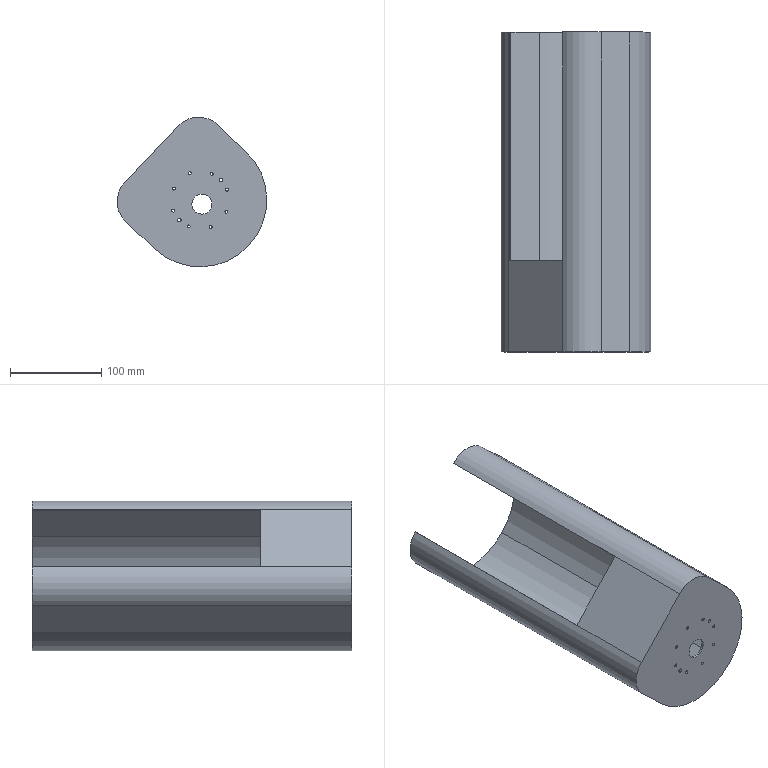Component | SolidWorks | ArmHousing3-1 | 1 solid | 42 faces | box 163.79 x 350 x 163.79 mm | volume 333891 mm3 | cylinder 30 | plane 12 | commonest cylinder face diameters 3.3 x16 4 x4 22 x2 146 x2 142 x2 56 x2 60 x2
build123d program:
from build123d import *

# Parameters (mm, degrees)
BOSS_EXTRUDE1_DEPTH     = 350
FILLET1_R               = 30
SHELL1_T                = -2
BOSS_EXTRUDE2_START     = -2
SKETCH3_R               = 1.65
SKETCH3_R_2             = 2
BOSS_EXTRUDE2_DEPTH     = 2
SKETCH4_W               = 250
SKETCH4_H               = 86
CUT_EXTRUDE1_2_DEPTH    = 2
CUT_EXTRUDE1_DEPTH      = 4
CUT_EXTRUDE1_DEPTH_BACK = 4
SKETCH1_R               = 11


with BuildPart() as part:
    # Sketch2 → Boss-Extrude1 (new body)
    with BuildSketch(Plane.XY):
        with BuildLine():
            Line((90, 148.39), (163, 148.39))
            Line((163, 148.39), (163, 294.39))
            Line((163, 294.39), (90, 294.39))
            ThreePointArc((90, 294.39), (17, 221.39), (90, 148.39))
        make_face()
    extrude(amount=BOSS_EXTRUDE1_DEPTH)

    # Fillet1
    fillet1_edges = [part.edges().sort_by_distance(p)[0] for p in [
        (163, 294.39, 175),
        (163, 148.39, 175),
    ]]
    fillet(fillet1_edges, radius=FILLET1_R)

    # Shell1
    shell1_openings = [part.faces().sort_by_distance(p)[0] for p in [
        (95.582, 221.39, 350),
        (95.582, 221.39, 0),
    ]]
    offset(amount=SHELL1_T, openings=shell1_openings, kind=Kind.INTERSECTION)

    # Sketch3 → Boss-Extrude2 (add)
    with BuildSketch(Plane(origin=(0, 0, 0), x_dir=(-1, 0, 0), z_dir=(0, 0, -1)).offset(BOSS_EXTRUDE2_START)):
        with BuildLine():
            Line((-90, 294.39), (-133, 294.39))
            ThreePointArc((-133, 294.39), (-154.213, 285.603), (-163, 264.39))
            Line((-163, 264.39), (-163, 178.39))
            ThreePointArc((-163, 178.39), (-154.213, 157.177), (-133, 148.39))
            Line((-133, 148.39), (-90, 148.39))
            ThreePointArc((-90, 148.39), (-17, 221.39), (-90, 294.39))
        make_face()
        with Locations((-61.491, 207.992)):
            Circle(SKETCH3_R, mode=Mode.SUBTRACT)
        with Locations((-79.315, 191.757)):
            Circle(SKETCH3_R, mode=Mode.SUBTRACT)
        with Locations((-60.368, 232.075)):
            Circle(SKETCH3_R, mode=Mode.SUBTRACT)
        with Locations((-76.602, 249.899)):
            Circle(SKETCH3_R, mode=Mode.SUBTRACT)
        with Locations((-88.532, 252.856)):
            Circle(SKETCH3_R_2, mode=Mode.SUBTRACT)
        with Locations((-100.685, 251.022)):
            Circle(SKETCH3_R, mode=Mode.SUBTRACT)
        with Locations((-91.468, 189.924)):
            Circle(SKETCH3_R_2, mode=Mode.SUBTRACT)
        with Locations((-103.398, 192.881)):
            Circle(SKETCH3_R, mode=Mode.SUBTRACT)
        with Locations((-119.632, 210.705)):
            Circle(SKETCH3_R, mode=Mode.SUBTRACT)
        with Locations((-118.509, 234.787)):
            Circle(SKETCH3_R, mode=Mode.SUBTRACT)
    extrude(amount=BOSS_EXTRUDE2_DEPTH)

    # Sketch4 → Cut-Extrude1_2 (cut)
    with BuildSketch(Plane(origin=(163, 0, 0), x_dir=(0, 0, -1), z_dir=(1, 0, 0))):
        with Locations((-225, 221.39)):
            Rectangle(SKETCH4_W, SKETCH4_H)
    extrude(amount=-CUT_EXTRUDE1_2_DEPTH, mode=Mode.SUBTRACT)

    # Sketch1 → Cut-Extrude1 (cut, two sides: drawn at the far end of the back side and taken through both)
    with BuildSketch(Plane.XY.offset(-CUT_EXTRUDE1_DEPTH_BACK)):
        with Locations(Location((85.6, 219.613, 0), (0, 0, 180))):
            Circle(SKETCH1_R)
    extrude(amount=CUT_EXTRUDE1_DEPTH + CUT_EXTRUDE1_DEPTH_BACK, mode=Mode.SUBTRACT)


solid = part.part

# Placed as in the assembly
solid = solid.moved(Location((499.474, 962, -2315.533), (-90, 0, -136.538)))